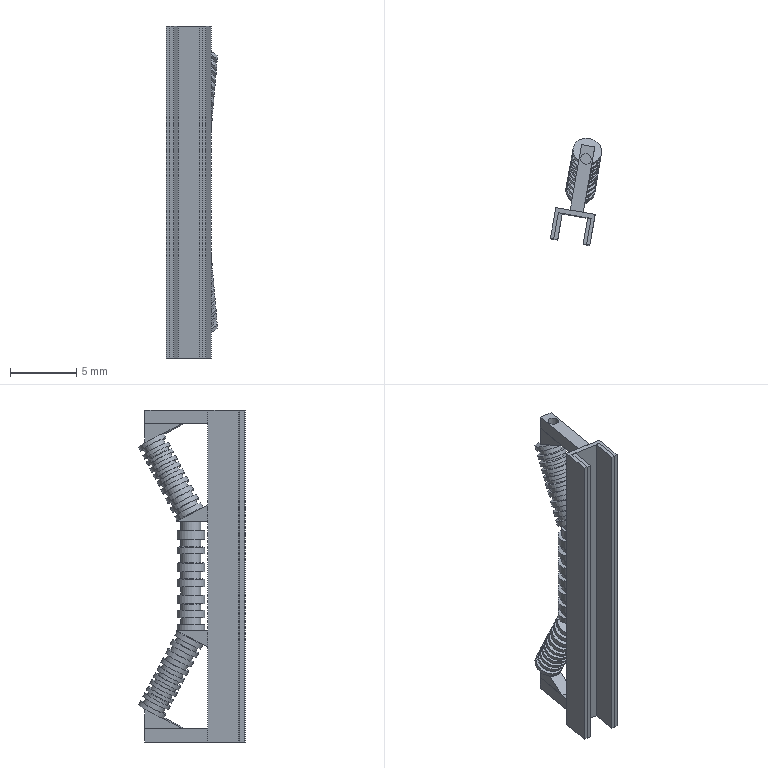Component | NX | H5_4 | 12 solids | 169 faces | volume 156 mm3 | cone 88 | plane 63 | cylinder 18 | commonest cylinder face diameters 2.065 x7 1.51 x7 0.8 x2 2.237 x2